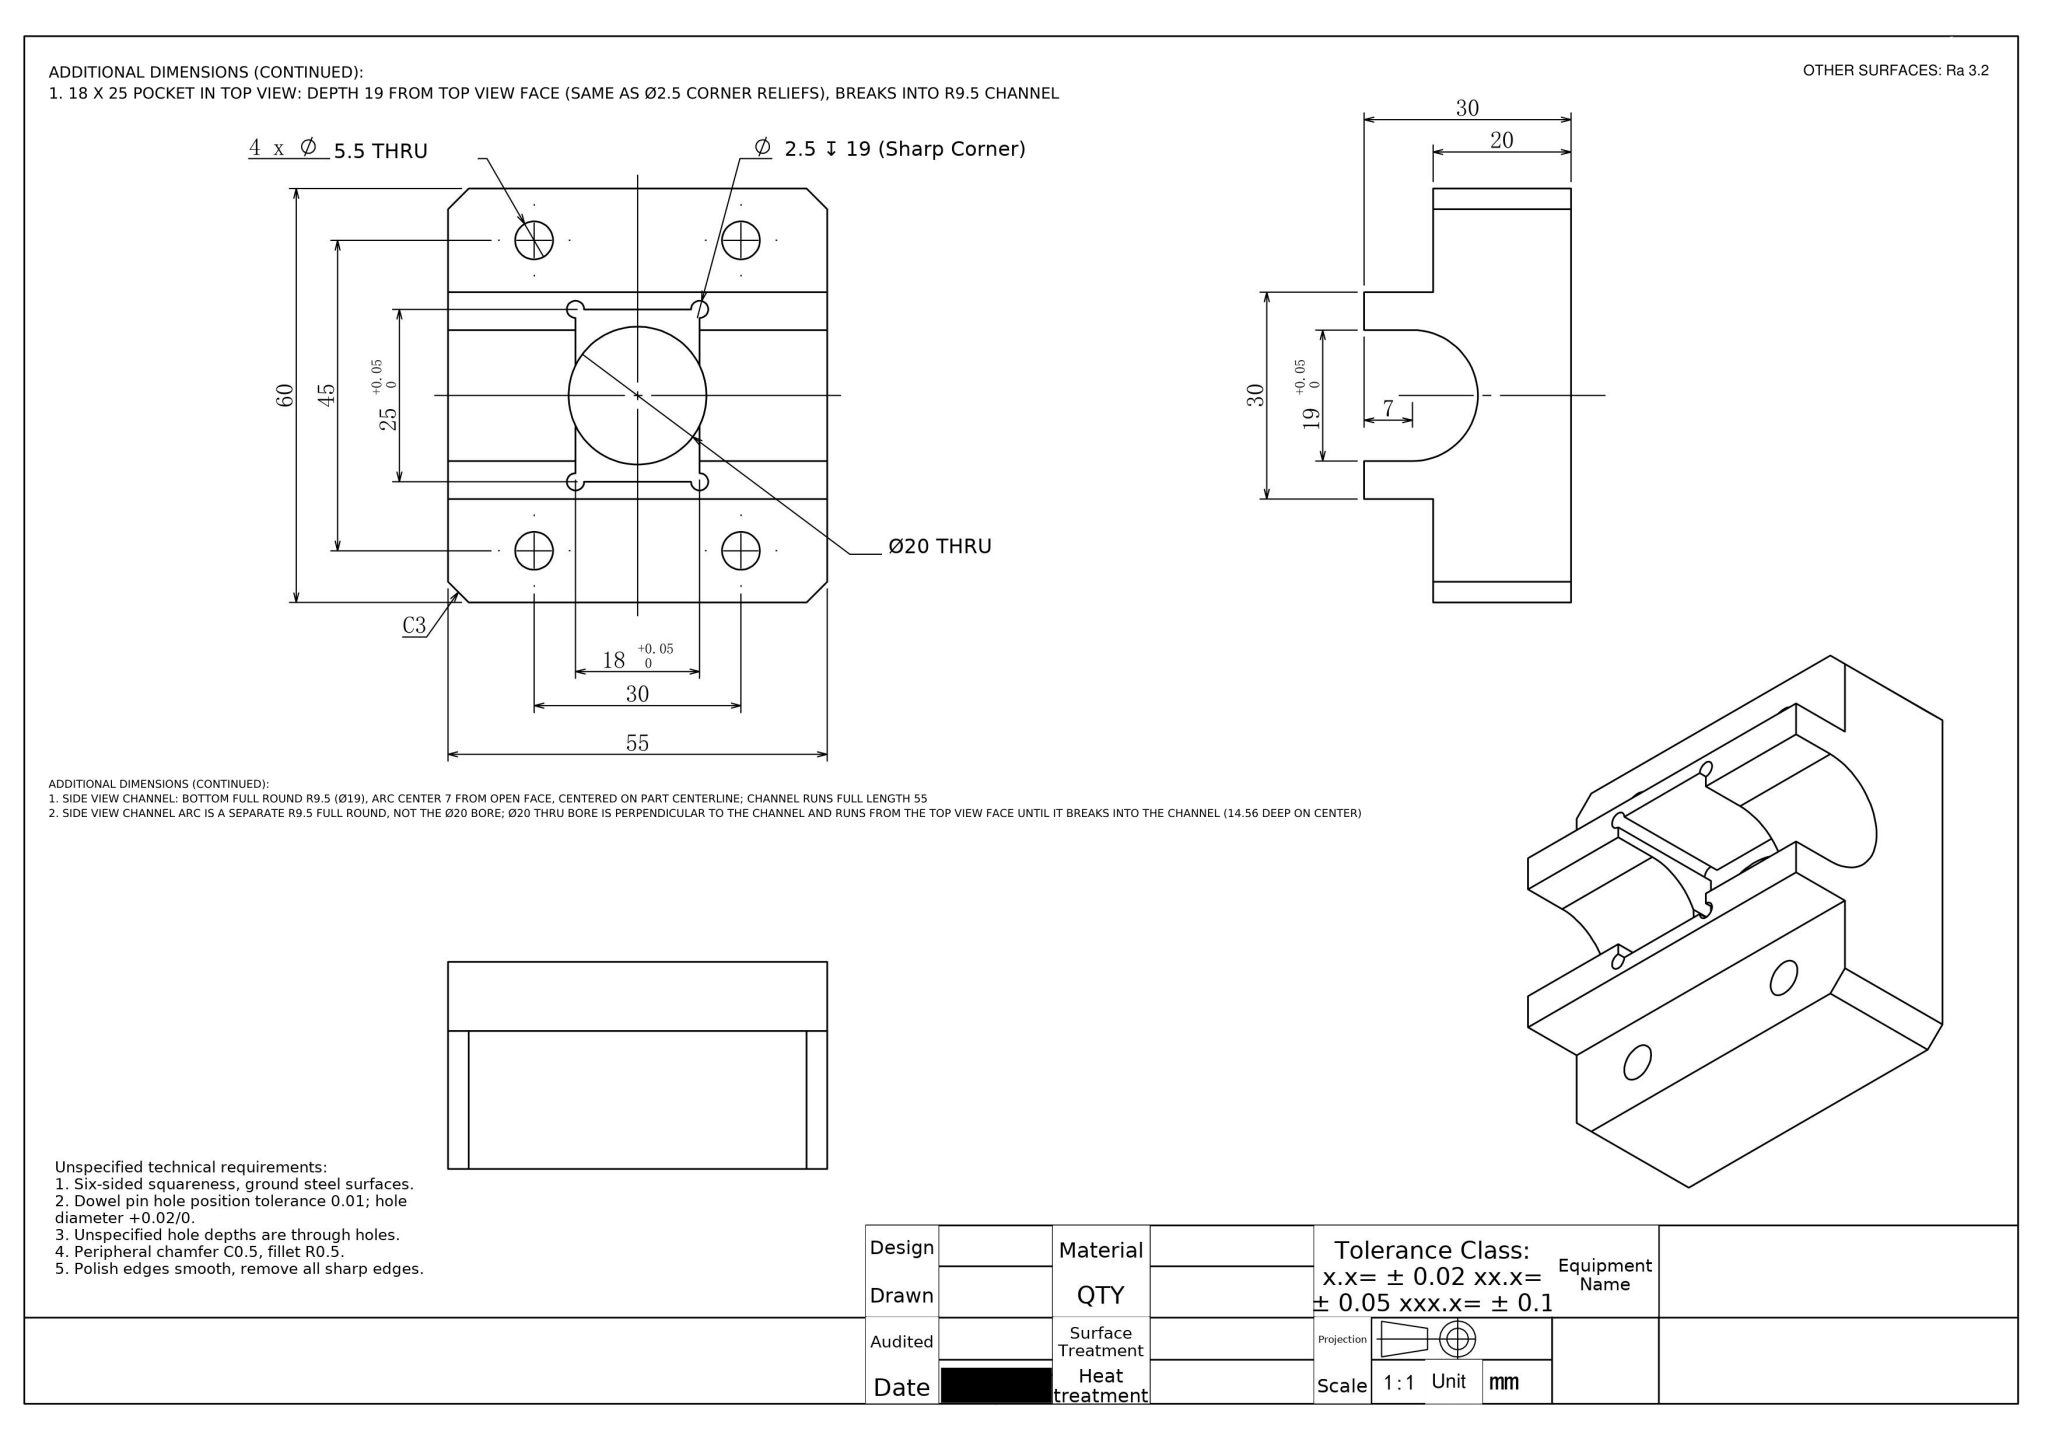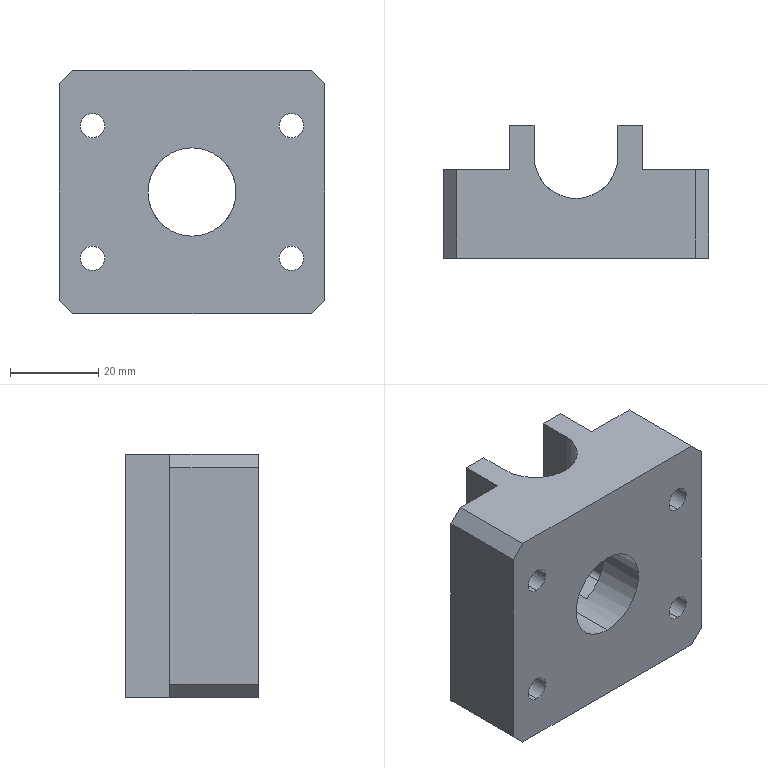Part | NX | mm | 1 solid | 45 faces | box 60 x 30 x 55 mm | volume 57756 mm3 | plane 27 | cylinder 18 | commonest cylinder face diameters 5.5 x8 2.5 x6 20 x2 19 x2